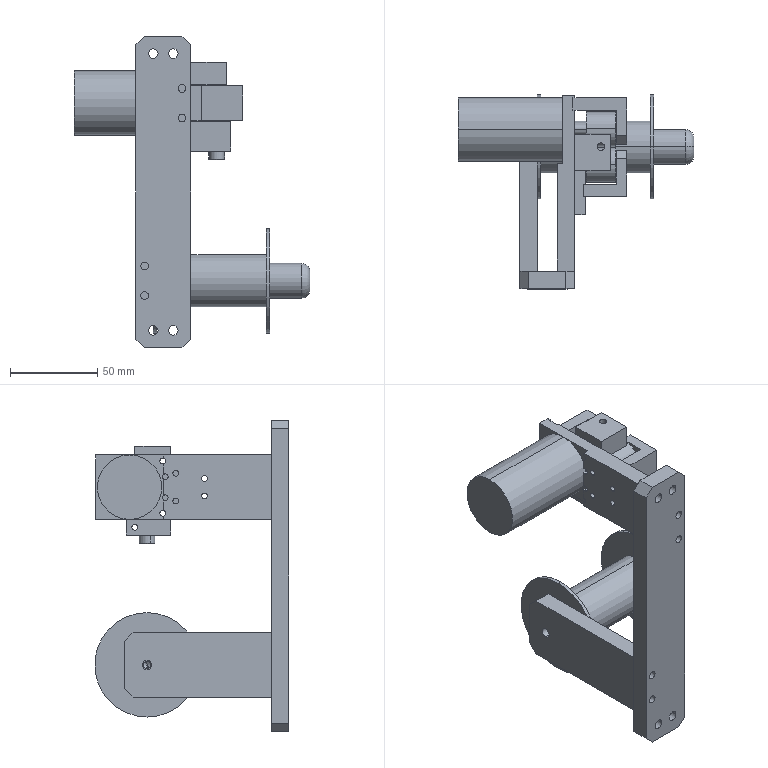Assembly | SolidWorks | mm | 14 component files | 14 solids | 297 faces | box 135.5 x 111.5 x 179 mm | volume 276290 mm3 | cylinder 149 | plane 122 | cone 20 | torus 6 | commonest cylinder face diameters 2.5 x22 3.3 x18 4.5 x16 3.5 x12 5.5 x10 8 x10 6 x10 20 x8
Bill of materials:
AS-011-JG0101 | 1 |  | Spool-shaped part: a cylindrical tube with a thin round flange at each end and a bore running through along the axis.
AS-011-JG0104 | 1 |  | Solid round rod with one end rounded or chamfered around its edge and a flat face in the middle of that end.
AS-011-JG0105 | 1 |  | Large cylindrical body with a stepped shaft coming out of one end face: a short boss of larger diameter, then a smaller round shaft. Six small holes are evenly spaced on a circle on an end face.
AS-011-JG0108 | 1 |  | Large solid cylinder with a thin, slightly larger collar step on one end face and a smaller coaxial cylindrical shaft extending from it.
AS-011-JG0129 | 1 |  | Long, thin, flat rectangular bar with all four corners chamfered and ten through holes: a pair of larger holes near each end and two pairs of smaller holes set along opposite long edges.
AS-011-JG0130 | 1 |  | L-shaped angle bracket. One leg has two chamfered corners at its free end, one large round hole and two smaller round holes. The other leg is a plain rectangular plate.
AS-011-JG0131 | 1 |  | Rectangular block plate with two obround slots, two small round holes and one larger round hole. A shallow step or groove runs across one face.
AS-011-JG0132 | 1 |  | L-shaped angle bracket with thicker legs. One leg has two chamfered corners, one large round hole and two smaller round holes. The other leg is a plain block.
AS-011-JG0133 | 1 |  | Symmetric large cylinder with a coaxial shaft coming out of each end face, with a thin shoulder collar between the body and each shaft.
AS-011-JG0134 | 1 |  | Flat rectangular plate or bar with two chamfered corners at one end and one small through hole near that end.
AS-011-JG0135 | 1 |  | Stepped cylindrical bushing-like part: a short, wider base flange and a longer, narrower cylindrical body, with chamfered edges and a small axial through hole.
AS-011-JG0136 | 1 |  | Rectangular plate with stepped thickness, a small notch or lip along one edge, one large round hole and twelve small round holes arranged in symmetric groups.
AS-011-JG0137 | 1 |  | Prismatic block with an L-shaped (stepped) profile. Two parallel round through-holes of different sizes, one in each section of the L. A narrow straight slit runs from an outer face into the larger hole, splitting the material around it like a clamp.
AS-011-JG0138 | 1 |  | Prismatic block with an L-shaped (stepped) profile. A larger round hole runs through the taller section, and a smaller round hole runs through on an axis at a right angle to it, through the top face of the overhanging extension.
Mates:
1. concentric | AS-011-JG0136-1 face at (-40, -18, -10) dir (1, 0, 0) r 6 | AS-011-JG0105-1 face at (-17, -18, -10) dir (1, 0, 0) r 18.5
2. concentric | AS-011-JG0136-1 face at (-40, -18, 5.5) dir (1, 0, 0) r 1.75 | AS-011-JG0105-1 face at (-37, -18, 5.5) dir (1, 0, 0) r 1.25
3. coincident | AS-011-JG0136-1 face at (-37, 1.5, -28.5) dir (-1, 0, 0) | AS-011-JG0105-1 face at (-37, 0.5, -10) dir (1, 0, 0)
4. concentric | AS-011-JG0130-1 face at (-42, -3.5, -16) dir (1, 0, 0) r 1.75 | AS-011-JG0136-1 face at (-40, -3.5, -16) dir (1, 0, 0) r 1.25
5. concentric | AS-011-JG0130-1 face at (-42, -3.5, -4) dir (1, 0, 0) r 1.75 | AS-011-JG0136-1 face at (-40, -3.5, -4) dir (1, 0, 0) r 1.25
6. coincident | AS-011-JG0130-1 face at (-31, -7, -20) dir (-1, 0, 0) | AS-011-JG0136-1 face at (-31, 0, -28.5) dir (1, 0, 0)
7. concentric | AS-011-JG0131-1 face at (-29, -38.5, -10) dir (1, 0, 0) r 7.5 | AS-011-JG0133-1 face at (-29.5, -38.5, -10) dir (-1, 0, 0) r 3
8. coincident | AS-011-JG0131-1 face at (-24, -30, 0) dir (1, 0, 0) | AS-011-JG0133-1 face at (-24, -34.5, -10) dir (-1, 0, 0)
9. concentric | AS-011-JG0131-1 face at (-30, -53, -4) dir (1, 0, 0) r 1.25 | AS-011-JG0132-1 face at (-25, -53, -4) dir (1, 0, 0) r 1.75
10. concentric | AS-011-JG0131-1 edge at (-30, -53, -16) dir (1, 0, 0) r 1.25 | AS-011-JG0132-1 face at (-25, -53, -16) dir (1, 0, 0) r 1.75
11. coincident | AS-011-JG0131-1 face at (-25, -30, 0) dir (1, 0, 0) | AS-011-JG0132-1 face at (-25, -56.5, -20) dir (-1, 0, 0)
12. coincident | AS-011-JG0131-1 face at (-30, -30, 0) dir (-1, 0, 0) | AS-011-JG0136-1 face at (-30, -99.5, 8.5) dir (1, 0, 0)
13. concentric | AS-011-JG0131-1 face at (-30, -61, -5) dir (1, 0, 0) r 2.25 | AS-011-JG0136-1 face at (-40, -61, -5) dir (1, 0, 0) r 1.65
14. concentric | AS-011-JG0131-1 face at (-30, -61, -15) dir (1, 0, 0) r 2.25 | AS-011-JG0136-1 face at (-40, -61, -15) dir (1, 0, 0) r 1.65
15. coincident | AS-011-JG0136-1 face at (-30, -99.5, 8.5) dir (1, 0, 0) | AS-011-JG0138-1 face at (-30, -21, 0.5) dir (-1, 0, 0)
16. concentric | AS-011-JG0136-1 face at (-40, -37, -25) dir (1, 0, 0) r 1.65 | AS-011-JG0137-1 face at (-17, -37, -25) dir (1, 0, 0) r 3.75
17. coincident | AS-011-JG0137-1 face at (-30, -41.5, -20.5) dir (0, -1, 0) | AS-011-JG0138-1 face at (-9.5, -41.5, 0.5) dir (0, -1, 0)
18. coincident | AS-011-JG0136-1 face at (-30, -99.5, 8.5) dir (1, 0, 0) | AS-011-JG0137-1 face at (-30, -41.5, -37.5) dir (-1, 0, 0)
19. concentric | AS-011-JG0135-1 face at (-15, -28, -23.5) dir (0, 0, 1) r 3.5 | AS-011-JG0137-1 face at (-15, -28, -37.5) dir (0, 0, 1) r 3.5
20. coincident | AS-011-JG0135-1 face at (-16.407, -24.795, -37.5) dir (0, 0, 1) | AS-011-JG0137-1 face at (-30, -16, -37.5) dir (0, 0, -1)
21. coincident | AS-011-JG0130-1 face at (-6, -7, -20) dir (-1, 0, 0) | AS-011-JG0108-1 face at (-6, -21.997, -9.843) dir (1, 0, 0)
22. concentric | AS-011-JG0105-1 face at (-17, -18, -10) dir (1, 0, 0) r 3 | AS-011-JG0108-1 face at (-42.5, -18, -10) dir (1, 0, 0) r 10
23. coincident | AS-011-JG0129-1 face at (-45.75, -99.5, -150.5) dir (0, 1, 0) | AS-011-JG0136-1 face at (-40, -99.5, 8.5) dir (0, -1, 0)
24. coincident | AS-011-JG0129-1 face at (-30, -99.5, -150.5) dir (1, 0, 0) | AS-011-JG0136-1 face at (-30, -99.5, 8.5) dir (1, 0, 0)
25. distance | AS-011-JG0129-1 face at (-45.75, -99.5, 28.5) dir (0, 0, 1) | AS-011-JG0136-1 face at (-40, 1.5, 8.5) dir (0, 0, 1)
26. coincident | AS-011-JG0129-1 face at (-45.75, -99.5, -150.5) dir (0, 1, 0) | AS-011-JG0134-1 face at (-51.5, -99.5, -93.5) dir (0, -1, 0)
27. coincident | AS-011-JG0129-1 face at (-61.5, -99.5, -150.5) dir (-1, 0, 0) | AS-011-JG0134-1 face at (-61.5, -15, -112) dir (-1, 0, 0)
28. distance | AS-011-JG0134-1 face at (-51.5, -20, -130.5) dir (0, 0, -1) | AS-011-JG0129-1 face at (-45.75, -99.5, -150.5) dir (0, 0, -1)
29. coincident | AS-011-JG0134-1 face at (-51.5, -15, -112) dir (1, 0, 0) | AS-011-JG0104-1 face at (-51.5, -28, -112) dir (-1, 0, 0)
30. concentric | AS-011-JG0134-1 face at (-51.5, -28, -112) dir (-1, 0, 0) r 2.75 | AS-011-JG0104-1 face at (38.5, -28, -112) dir (-1, 0, 0) r 10
31. concentric | AS-011-JG0136-1 face at (-40, -37, 5) dir (1, 0, 0) r 1.65 | AS-011-JG0138-1 face at (-32.5, -37, 5) dir (1, 0, 0) r 2.25
32. concentric | AS-011-JG0104-1 face at (38.5, -28, -112) dir (-1, 0, 0) r 10 | AS-011-JG0101-2 face at (-51.5, -28, -112) dir (-1, 0, 0) r 15
33. coincident | AS-011-JG0134-1 face at (-51.5, -15, -112) dir (1, 0, 0) | AS-011-JG0101-2 face at (-51.5, -18, -112.002) dir (-1, 0, 0)